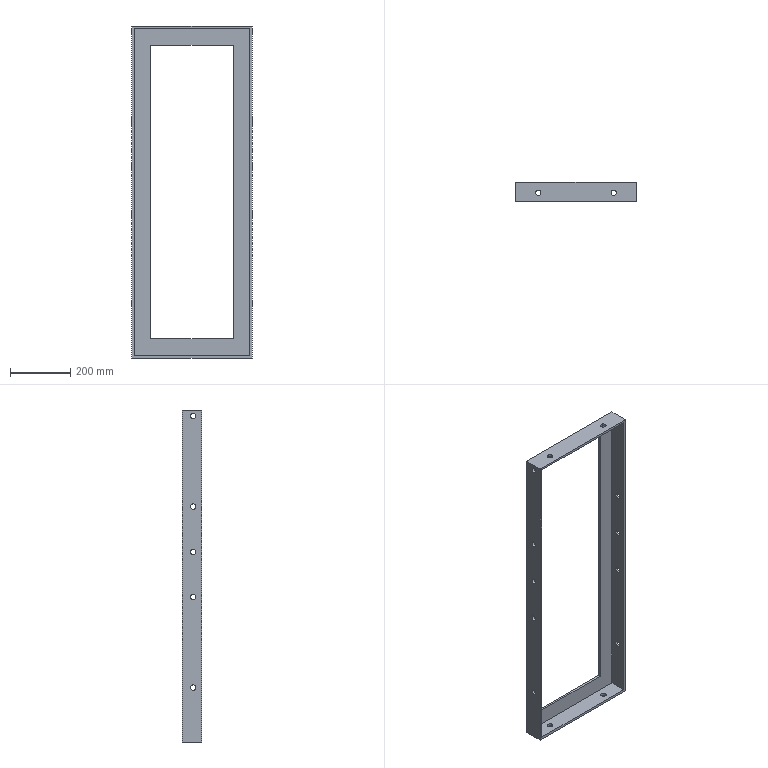Component | SolidWorks | GuideFrame_2-1 | 1 solid | 43 faces | box 400 x 63 x 1100 mm | volume 2662411 mm3 | cylinder 28 | plane 15 | commonest cylinder face diameters 18 x28
build123d program:
from build123d import *

# Parameters (mm, degrees)
SKETCH1_W                 = 400
SKETCH1_H                 = 1100
BOSS_EXTRUDE1_DEPTH       = 63
SKETCH2_W                 = 384
SKETCH2_H                 = 1084
CUT_EXTRUDE1_DEPTH        = 55
SKETCH3_W                 = 274
SKETCH3_H                 = 974
CUT_EXTRUDE2_DEPTH        = 8
SIZE_MM_DOWEL_PIN_HOLE0_D = 18
SIZE_MM_DOWEL_PIN_HOLE1_D = 18


with BuildPart() as part:
    # Sketch1 → Boss-Extrude1 (new body)
    with BuildSketch(Plane.XY):
        Rectangle(SKETCH1_W, SKETCH1_H)
    extrude(amount=BOSS_EXTRUDE1_DEPTH)

    # Sketch2 → Cut-Extrude1 (cut)
    with BuildSketch(Plane.XY.offset(63)):
        Rectangle(SKETCH2_W, SKETCH2_H)
    extrude(amount=-CUT_EXTRUDE1_DEPTH, mode=Mode.SUBTRACT)

    # Sketch3 → Cut-Extrude2 (cut)
    with BuildSketch(Plane.XY.offset(8)):
        Rectangle(SKETCH3_W, SKETCH3_H)
    extrude(amount=-CUT_EXTRUDE2_DEPTH, mode=Mode.SUBTRACT)

    # Size mm Dowel Pin Hole0 (through all)
    with Locations(Plane(origin=(0, 550, 0), x_dir=(1, 0, 0), z_dir=(0, 1, 0))):
        with Locations((-125, -35), (125, -35)):
            Hole(SIZE_MM_DOWEL_PIN_HOLE0_D / 2)

    # Size mm Dowel Pin Hole1 (through all)
    with Locations(Plane.ZY.offset(200)):
        with Locations((35, 530), (35, 230), (35, 80), (35, -70), (35, -370)):
            Hole(SIZE_MM_DOWEL_PIN_HOLE1_D / 2)


solid = part.part

# Placed as in the assembly
solid = solid.moved(Location((0, -290, -80), (90, 0, 0)))